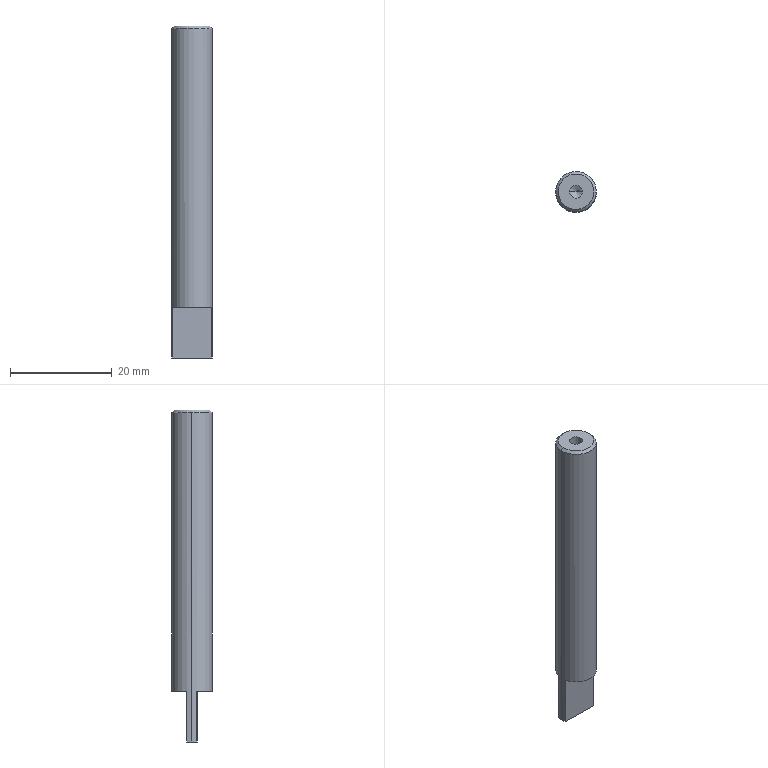Component | SolidWorks | 002MaterialPickingModuleA-1_004SidePlugModule-1_J-010-1 | 1 solid | 14 faces | box 8 x 8 x 65.25 mm | volume 2894 mm3 | plane 6 | cone 4 | cylinder 4 | commonest cylinder face diameters 2.5 x2 8 x2 | material 45
build123d program:
from build123d import *

# Parameters (mm, degrees)
SKETCH1_R             = 4
BOSS_EXTRUDE1_DEPTH   = 65.25
CUT_EXTRUDE1_START    = -10
CUT_EXTRUDE1_DEPTH    = 10
M3_TAPPED_HOLE1_D     = 2.5
M3_TAPPED_HOLE1_DEPTH = 7.5
M3_TAPPED_HOLE1_TIP   = 0.7511
CHAMFER1_SIZE         = 0.5


with BuildPart() as part:
    # Sketch1 → Boss-Extrude1 (new body)
    with BuildSketch(Plane.XY):
        Circle(SKETCH1_R)
    extrude(amount=BOSS_EXTRUDE1_DEPTH)

    # Sketch2 → Cut-Extrude1 (cut)
    with BuildSketch(Plane.XY.offset(65.25).offset(CUT_EXTRUDE1_START)):
        with BuildLine():
            Line((3.873, -1), (-3.873, -1))
            ThreePointArc((-3.873, -1), (0, -4), (3.873, -1))
        make_face()
        with BuildLine():
            Line((3.873, 1), (-3.873, 1))
            ThreePointArc((-3.873, 1), (0, 4), (3.873, 1))
        make_face()
    extrude(amount=CUT_EXTRUDE1_DEPTH, mode=Mode.SUBTRACT)

    # M3 Tapped Hole1
    with Locations(Plane(origin=(0, 0, 0), x_dir=(-1, 0, 0), z_dir=(0, 0, -1))):
        with Locations((0, 0)):
            Hole(M3_TAPPED_HOLE1_D / 2, depth=M3_TAPPED_HOLE1_DEPTH)
            with Locations((0, 0, -(M3_TAPPED_HOLE1_DEPTH + M3_TAPPED_HOLE1_TIP / 2))):  # 118° drill point
                Cone(0, M3_TAPPED_HOLE1_D / 2, M3_TAPPED_HOLE1_TIP, mode=Mode.SUBTRACT)

    # Chamfer1
    chamfer1_edges = [part.edges().sort_by_distance(p)[0] for p in [
        (-4, 0, 0),
    ]]
    chamfer(chamfer1_edges, length=CHAMFER1_SIZE)


solid = part.part

# Placed as in the assembly
solid = solid.moved(Location((70.325, 296.019, 469.581), (-180, 0, -179.039)))
STEP:
#1=CARTESIAN_POINT('',(2.906,11.652,18.487));
#2=VERTEX_POINT('',#1);
#3=CARTESIAN_POINT('',(2.631,11.657,18.487));
#4=VERTEX_POINT('',#3);
#5=CARTESIAN_POINT('',(2.769,11.654,18.487));
#6=DIRECTION('',(0.,0.,1.));
#7=DIRECTION('',(-0.9999,0.01678,0.));
#8=AXIS2_PLACEMENT_3D('',#5,#6,#7);
#9=CIRCLE('',#8,0.1378);
#10=EDGE_CURVE('',#2,#4,#9,.T.);
#11=ORIENTED_EDGE('',*,*,#10,.F.);
#12=CARTESIAN_POINT('',(2.926,11.652,18.468));
#13=VERTEX_POINT('',#12);
#14=CARTESIAN_POINT('',(2.926,11.652,18.468));
#15=DIRECTION('',(0.707,-0.01187,-0.7071));
#16=VECTOR('',#15,39.37);
#17=LINE('',#14,#16);
#18=EDGE_CURVE('',#2,#13,#17,.T.);
#19=ORIENTED_EDGE('',*,*,#18,.T.);
#20=CARTESIAN_POINT('',(2.611,11.657,18.468));
#21=VERTEX_POINT('',#20);
#22=CARTESIAN_POINT('',(2.769,11.654,18.468));
#23=DIRECTION('',(0.,0.,-1.));
#24=DIRECTION('',(-0.9999,0.01678,0.));
#25=AXIS2_PLACEMENT_3D('',#22,#23,#24);
#26=CIRCLE('',#25,0.1575);
#27=EDGE_CURVE('',#21,#13,#26,.T.);
#28=ORIENTED_EDGE('',*,*,#27,.F.);
#29=CARTESIAN_POINT('',(2.611,11.657,18.468));
#30=DIRECTION('',(-0.707,0.01187,-0.7071));
#31=VECTOR('',#30,39.37);
#32=LINE('',#29,#31);
#33=EDGE_CURVE('',#4,#21,#32,.T.);
#34=ORIENTED_EDGE('',*,*,#33,.F.);
#35=EDGE_LOOP('',(#11,#19,#28,#34));
#36=FACE_OUTER_BOUND('',#35,.T.);
#37=CARTESIAN_POINT('',(2.769,11.654,18.468));
#38=DIRECTION('',(0.,0.,-1.));
#39=DIRECTION('',(-0.9999,0.01678,0.));
#40=AXIS2_PLACEMENT_3D('',#37,#38,#39);
#41=CONICAL_SURFACE('',#40,0.1575,0.7854);
#42=ADVANCED_FACE('',(#36),#41,.T.);
#43=CARTESIAN_POINT('',(2.719,11.655,18.192));
#44=VERTEX_POINT('',#43);
#45=CARTESIAN_POINT('',(2.818,11.653,18.192));
#46=VERTEX_POINT('',#45);
#47=CARTESIAN_POINT('',(2.769,11.654,18.192));
#48=DIRECTION('',(0.,0.,1.));
#49=DIRECTION('',(0.9999,-0.01678,0.));
#50=AXIS2_PLACEMENT_3D('',#47,#48,#49);
#51=CIRCLE('',#50,0.04921);
#52=EDGE_CURVE('',#44,#46,#51,.T.);
#53=ORIENTED_EDGE('',*,*,#52,.F.);
#54=CARTESIAN_POINT('',(2.719,11.655,18.487));
#55=VERTEX_POINT('',#54);
#56=CARTESIAN_POINT('',(2.719,11.655,18.487));
#57=DIRECTION('',(0.,0.,1.));
#58=VECTOR('',#57,39.37);
#59=LINE('',#56,#58);
#60=EDGE_CURVE('',#44,#55,#59,.T.);
#61=ORIENTED_EDGE('',*,*,#60,.T.);
#62=CARTESIAN_POINT('',(2.818,11.653,18.487));
#63=VERTEX_POINT('',#62);
#64=CARTESIAN_POINT('',(2.769,11.654,18.487));
#65=DIRECTION('',(0.,0.,1.));
#66=DIRECTION('',(0.9999,-0.01678,0.));
#67=AXIS2_PLACEMENT_3D('',#64,#65,#66);
#68=CIRCLE('',#67,0.04921);
#69=EDGE_CURVE('',#55,#63,#68,.T.);
#70=ORIENTED_EDGE('',*,*,#69,.T.);
#71=CARTESIAN_POINT('',(2.818,11.653,18.487));
#72=DIRECTION('',(0.,0.,1.));
#73=VECTOR('',#72,39.37);
#74=LINE('',#71,#73);
#75=EDGE_CURVE('',#46,#63,#74,.T.);
#76=ORIENTED_EDGE('',*,*,#75,.F.);
#77=EDGE_LOOP('',(#53,#61,#70,#76));
#78=FACE_OUTER_BOUND('',#77,.T.);
#79=CARTESIAN_POINT('',(2.769,11.654,18.487));
#80=DIRECTION('',(0.,0.,1.));
#81=DIRECTION('',(0.9999,-0.01678,0.));
#82=AXIS2_PLACEMENT_3D('',#79,#80,#81);
#83=CYLINDRICAL_SURFACE('',#82,0.04921);
#84=ADVANCED_FACE('',(#78),#83,.F.);
#85=CARTESIAN_POINT('',(2.769,11.654,18.163));
#86=VERTEX_POINT('',#85);
#87=CARTESIAN_POINT('',(2.818,11.653,18.192));
#88=DIRECTION('',(0.857,-0.01438,0.515));
#89=VECTOR('',#88,39.37);
#90=LINE('',#87,#89);
#91=EDGE_CURVE('',#86,#46,#90,.T.);
#92=ORIENTED_EDGE('',*,*,#91,.F.);
#93=CARTESIAN_POINT('',(2.719,11.655,18.192));
#94=DIRECTION('',(-0.857,0.01438,0.515));
#95=VECTOR('',#94,39.37);
#96=LINE('',#93,#95);
#97=EDGE_CURVE('',#86,#44,#96,.T.);
#98=ORIENTED_EDGE('',*,*,#97,.T.);
#99=ORIENTED_EDGE('',*,*,#52,.T.);
#100=EDGE_LOOP('',(#92,#98,#99));
#101=FACE_OUTER_BOUND('',#100,.T.);
#102=CARTESIAN_POINT('',(2.769,11.654,18.192));
#103=DIRECTION('',(0.,0.,1.));
#104=DIRECTION('',(0.9999,-0.01678,0.));
#105=AXIS2_PLACEMENT_3D('',#102,#103,#104);
#106=CONICAL_SURFACE('',#105,0.04921,1.03);
#107=ADVANCED_FACE('',(#101),#106,.F.);
#108=CARTESIAN_POINT('',(2.611,11.657,15.919));
#109=VERTEX_POINT('',#108);
#110=CARTESIAN_POINT('',(2.617,11.696,15.919));
#111=VERTEX_POINT('',#110);
#112=CARTESIAN_POINT('',(2.769,11.654,15.919));
#113=DIRECTION('',(0.,0.,-1.));
#114=DIRECTION('',(-0.9999,0.01678,0.));
#115=AXIS2_PLACEMENT_3D('',#112,#113,#114);
#116=CIRCLE('',#115,0.1575);
#117=EDGE_CURVE('',#109,#111,#116,.T.);
#118=ORIENTED_EDGE('',*,*,#117,.F.);
#119=CARTESIAN_POINT('',(2.611,11.657,15.919));
#120=DIRECTION('',(0.,0.,1.));
#121=VECTOR('',#120,39.37);
#122=LINE('',#119,#121);
#123=EDGE_CURVE('',#109,#21,#122,.T.);
#124=ORIENTED_EDGE('',*,*,#123,.T.);
#125=ORIENTED_EDGE('',*,*,#27,.T.);
#126=CARTESIAN_POINT('',(2.926,11.652,15.919));
#127=VERTEX_POINT('',#126);
#128=CARTESIAN_POINT('',(2.926,11.652,15.919));
#129=DIRECTION('',(0.,0.,1.));
#130=VECTOR('',#129,39.37);
#131=LINE('',#128,#130);
#132=EDGE_CURVE('',#127,#13,#131,.T.);
#133=ORIENTED_EDGE('',*,*,#132,.F.);
#134=CARTESIAN_POINT('',(2.922,11.691,15.919));
#135=VERTEX_POINT('',#134);
#136=CARTESIAN_POINT('',(2.769,11.654,15.919));
#137=DIRECTION('',(0.,0.,-1.));
#138=DIRECTION('',(-0.9999,0.01678,0.));
#139=AXIS2_PLACEMENT_3D('',#136,#137,#138);
#140=CIRCLE('',#139,0.1575);
#141=EDGE_CURVE('',#135,#127,#140,.T.);
#142=ORIENTED_EDGE('',*,*,#141,.F.);
#143=CARTESIAN_POINT('',(2.922,11.691,16.312));
#144=VERTEX_POINT('',#143);
#145=CARTESIAN_POINT('',(2.922,11.691,16.312));
#146=DIRECTION('',(0.,0.,-1.));
#147=VECTOR('',#146,39.37);
#148=LINE('',#145,#147);
#149=EDGE_CURVE('',#144,#135,#148,.T.);
#150=ORIENTED_EDGE('',*,*,#149,.F.);
#151=CARTESIAN_POINT('',(2.617,11.696,16.312));
#152=VERTEX_POINT('',#151);
#153=CARTESIAN_POINT('',(2.769,11.654,16.312));
#154=DIRECTION('',(0.,0.,-1.));
#155=DIRECTION('',(-0.9999,0.01678,0.));
#156=AXIS2_PLACEMENT_3D('',#153,#154,#155);
#157=CIRCLE('',#156,0.1575);
#158=EDGE_CURVE('',#152,#144,#157,.T.);
#159=ORIENTED_EDGE('',*,*,#158,.F.);
#160=CARTESIAN_POINT('',(2.617,11.696,16.312));
#161=DIRECTION('',(0.,0.,-1.));
#162=VECTOR('',#161,39.37);
#163=LINE('',#160,#162);
#164=EDGE_CURVE('',#152,#111,#163,.T.);
#165=ORIENTED_EDGE('',*,*,#164,.T.);
#166=EDGE_LOOP('',(#118,#124,#125,#133,#142,#150,#159,#165));
#167=FACE_OUTER_BOUND('',#166,.T.);
#168=CARTESIAN_POINT('',(2.769,11.654,15.919));
#169=DIRECTION('',(0.,0.,1.));
#170=DIRECTION('',(0.9999,-0.01678,0.));
#171=AXIS2_PLACEMENT_3D('',#168,#169,#170);
#172=CYLINDRICAL_SURFACE('',#171,0.1575);
#173=ADVANCED_FACE('',(#167),#172,.T.);
#174=ORIENTED_EDGE('',*,*,#123,.F.);
#175=CARTESIAN_POINT('',(2.616,11.617,15.919));
#176=VERTEX_POINT('',#175);
#177=CARTESIAN_POINT('',(2.769,11.654,15.919));
#178=DIRECTION('',(0.,0.,-1.));
#179=DIRECTION('',(-0.9999,0.01678,0.));
#180=AXIS2_PLACEMENT_3D('',#177,#178,#179);
#181=CIRCLE('',#180,0.1575);
#182=EDGE_CURVE('',#176,#109,#181,.T.);
#183=ORIENTED_EDGE('',*,*,#182,.F.);
#184=CARTESIAN_POINT('',(2.616,11.617,16.312));
#185=VERTEX_POINT('',#184);
#186=CARTESIAN_POINT('',(2.616,11.617,16.312));
#187=DIRECTION('',(0.,0.,-1.));
#188=VECTOR('',#187,39.37);
#189=LINE('',#186,#188);
#190=EDGE_CURVE('',#185,#176,#189,.T.);
#191=ORIENTED_EDGE('',*,*,#190,.F.);
#192=CARTESIAN_POINT('',(2.92,11.612,16.312));
#193=VERTEX_POINT('',#192);
#194=CARTESIAN_POINT('',(2.769,11.654,16.312));
#195=DIRECTION('',(0.,0.,-1.));
#196=DIRECTION('',(-0.9999,0.01678,0.));
#197=AXIS2_PLACEMENT_3D('',#194,#195,#196);
#198=CIRCLE('',#197,0.1575);
#199=EDGE_CURVE('',#193,#185,#198,.T.);
#200=ORIENTED_EDGE('',*,*,#199,.F.);
#201=CARTESIAN_POINT('',(2.92,11.612,15.919));
#202=VERTEX_POINT('',#201);
#203=CARTESIAN_POINT('',(2.92,11.612,16.312));
#204=DIRECTION('',(0.,0.,-1.));
#205=VECTOR('',#204,39.37);
#206=LINE('',#203,#205);
#207=EDGE_CURVE('',#193,#202,#206,.T.);
#208=ORIENTED_EDGE('',*,*,#207,.T.);
#209=CARTESIAN_POINT('',(2.769,11.654,15.919));
#210=DIRECTION('',(0.,0.,-1.));
#211=DIRECTION('',(-0.9999,0.01678,0.));
#212=AXIS2_PLACEMENT_3D('',#209,#210,#211);
#213=CIRCLE('',#212,0.1575);
#214=EDGE_CURVE('',#127,#202,#213,.T.);
#215=ORIENTED_EDGE('',*,*,#214,.F.);
#216=ORIENTED_EDGE('',*,*,#132,.T.);
#217=CARTESIAN_POINT('',(2.769,11.654,18.468));
#218=DIRECTION('',(0.,0.,-1.));
#219=DIRECTION('',(-0.9999,0.01678,0.));
#220=AXIS2_PLACEMENT_3D('',#217,#218,#219);
#221=CIRCLE('',#220,0.1575);
#222=EDGE_CURVE('',#13,#21,#221,.T.);
#223=ORIENTED_EDGE('',*,*,#222,.T.);
#224=EDGE_LOOP('',(#174,#183,#191,#200,#208,#215,#216,#223));
#225=FACE_OUTER_BOUND('',#224,.T.);
#226=CARTESIAN_POINT('',(2.769,11.654,15.919));
#227=DIRECTION('',(0.,0.,1.));
#228=DIRECTION('',(0.9999,-0.01678,0.));
#229=AXIS2_PLACEMENT_3D('',#226,#227,#228);
#230=CYLINDRICAL_SURFACE('',#229,0.1575);
#231=ADVANCED_FACE('',(#225),#230,.T.);
#232=CARTESIAN_POINT('',(2.616,11.617,15.919));
#233=DIRECTION('',(0.9999,-0.01678,0.));
#234=VECTOR('',#233,39.37);
#235=LINE('',#232,#234);
#236=EDGE_CURVE('',#176,#202,#235,.T.);
#237=ORIENTED_EDGE('',*,*,#236,.F.);
#238=ORIENTED_EDGE('',*,*,#182,.T.);
#239=ORIENTED_EDGE('',*,*,#117,.T.);
#240=CARTESIAN_POINT('',(2.617,11.696,15.919));
#241=DIRECTION('',(-0.9999,0.01678,0.));
#242=VECTOR('',#241,39.37);
#243=LINE('',#240,#242);
#244=EDGE_CURVE('',#135,#111,#243,.T.);
#245=ORIENTED_EDGE('',*,*,#244,.F.);
#246=ORIENTED_EDGE('',*,*,#141,.T.);
#247=ORIENTED_EDGE('',*,*,#214,.T.);
#248=EDGE_LOOP('',(#237,#238,#239,#245,#246,#247));
#249=FACE_OUTER_BOUND('',#248,.T.);
#250=CARTESIAN_POINT('',(2.769,11.654,15.919));
#251=DIRECTION('',(0.,0.,-1.));
#252=DIRECTION('',(-0.9999,0.01678,0.));
#253=AXIS2_PLACEMENT_3D('',#250,#251,#252);
#254=PLANE('',#253);
#255=ADVANCED_FACE('',(#249),#254,.T.);
#256=CARTESIAN_POINT('',(2.769,11.654,18.487));
#257=DIRECTION('',(0.,0.,1.));
#258=DIRECTION('',(-0.9999,0.01678,0.));
#259=AXIS2_PLACEMENT_3D('',#256,#257,#258);
#260=CIRCLE('',#259,0.1378);
#261=EDGE_CURVE('',#4,#2,#260,.T.);
#262=ORIENTED_EDGE('',*,*,#261,.T.);
#263=ORIENTED_EDGE('',*,*,#10,.T.);
#264=EDGE_LOOP('',(#262,#263));
#265=FACE_OUTER_BOUND('',#264,.T.);
#266=CARTESIAN_POINT('',(2.769,11.654,18.487));
#267=DIRECTION('',(0.,0.,1.));
#268=DIRECTION('',(0.9999,-0.01678,0.));
#269=AXIS2_PLACEMENT_3D('',#266,#267,#268);
#270=CIRCLE('',#269,0.04921);
#271=EDGE_CURVE('',#63,#55,#270,.T.);
#272=ORIENTED_EDGE('',*,*,#271,.F.);
#273=ORIENTED_EDGE('',*,*,#69,.F.);
#274=EDGE_LOOP('',(#272,#273));
#275=FACE_BOUND('',#274,.T.);
#276=CARTESIAN_POINT('',(2.769,11.654,18.487));
#277=DIRECTION('',(0.,0.,-1.));
#278=DIRECTION('',(-0.9999,0.01678,0.));
#279=AXIS2_PLACEMENT_3D('',#276,#277,#278);
#280=PLANE('',#279);
#281=ADVANCED_FACE('',(#265,#275),#280,.F.);
#282=ORIENTED_EDGE('',*,*,#244,.T.);
#283=ORIENTED_EDGE('',*,*,#164,.F.);
#284=CARTESIAN_POINT('',(2.617,11.696,16.312));
#285=DIRECTION('',(-0.9999,0.01678,0.));
#286=VECTOR('',#285,39.37);
#287=LINE('',#284,#286);
#288=EDGE_CURVE('',#144,#152,#287,.T.);
#289=ORIENTED_EDGE('',*,*,#288,.F.);
#290=ORIENTED_EDGE('',*,*,#149,.T.);
#291=EDGE_LOOP('',(#282,#283,#289,#290));
#292=FACE_OUTER_BOUND('',#291,.T.);
#293=CARTESIAN_POINT('',(2.617,11.696,16.312));
#294=DIRECTION('',(-0.01678,-0.9999,0.));
#295=DIRECTION('',(0.,0.,1.));
#296=AXIS2_PLACEMENT_3D('',#293,#294,#295);
#297=PLANE('',#296);
#298=ADVANCED_FACE('',(#292),#297,.F.);
#299=ORIENTED_EDGE('',*,*,#158,.T.);
#300=ORIENTED_EDGE('',*,*,#288,.T.);
#301=EDGE_LOOP('',(#299,#300));
#302=FACE_OUTER_BOUND('',#301,.T.);
#303=CARTESIAN_POINT('',(2.769,11.654,16.312));
#304=DIRECTION('',(0.,0.,-1.));
#305=DIRECTION('',(-0.9999,0.01678,0.));
#306=AXIS2_PLACEMENT_3D('',#303,#304,#305);
#307=PLANE('',#306);
#308=ADVANCED_FACE('',(#302),#307,.T.);
#309=ORIENTED_EDGE('',*,*,#236,.T.);
#310=ORIENTED_EDGE('',*,*,#207,.F.);
#311=CARTESIAN_POINT('',(2.616,11.617,16.312));
#312=DIRECTION('',(0.9999,-0.01678,0.));
#313=VECTOR('',#312,39.37);
#314=LINE('',#311,#313);
#315=EDGE_CURVE('',#185,#193,#314,.T.);
#316=ORIENTED_EDGE('',*,*,#315,.F.);
#317=ORIENTED_EDGE('',*,*,#190,.T.);
#318=EDGE_LOOP('',(#309,#310,#316,#317));
#319=FACE_OUTER_BOUND('',#318,.T.);
#320=CARTESIAN_POINT('',(2.616,11.617,16.312));
#321=DIRECTION('',(0.01678,0.9999,0.));
#322=DIRECTION('',(0.,0.,-1.));
#323=AXIS2_PLACEMENT_3D('',#320,#321,#322);
#324=PLANE('',#323);
#325=ADVANCED_FACE('',(#319),#324,.F.);
#326=ORIENTED_EDGE('',*,*,#199,.T.);
#327=ORIENTED_EDGE('',*,*,#315,.T.);
#328=EDGE_LOOP('',(#326,#327));
#329=FACE_OUTER_BOUND('',#328,.T.);
#330=CARTESIAN_POINT('',(2.769,11.654,16.312));
#331=DIRECTION('',(0.,0.,-1.));
#332=DIRECTION('',(-0.9999,0.01678,0.));
#333=AXIS2_PLACEMENT_3D('',#330,#331,#332);
#334=PLANE('',#333);
#335=ADVANCED_FACE('',(#329),#334,.T.);
#336=ORIENTED_EDGE('',*,*,#97,.F.);
#337=ORIENTED_EDGE('',*,*,#91,.T.);
#338=CARTESIAN_POINT('',(2.769,11.654,18.192));
#339=DIRECTION('',(0.,0.,1.));
#340=DIRECTION('',(0.9999,-0.01678,0.));
#341=AXIS2_PLACEMENT_3D('',#338,#339,#340);
#342=CIRCLE('',#341,0.04921);
#343=EDGE_CURVE('',#46,#44,#342,.T.);
#344=ORIENTED_EDGE('',*,*,#343,.T.);
#345=EDGE_LOOP('',(#336,#337,#344));
#346=FACE_OUTER_BOUND('',#345,.T.);
#347=CARTESIAN_POINT('',(2.769,11.654,18.192));
#348=DIRECTION('',(0.,0.,1.));
#349=DIRECTION('',(0.9999,-0.01678,0.));
#350=AXIS2_PLACEMENT_3D('',#347,#348,#349);
#351=CONICAL_SURFACE('',#350,0.04921,1.03);
#352=ADVANCED_FACE('',(#346),#351,.F.);
#353=ORIENTED_EDGE('',*,*,#60,.F.);
#354=ORIENTED_EDGE('',*,*,#343,.F.);
#355=ORIENTED_EDGE('',*,*,#75,.T.);
#356=ORIENTED_EDGE('',*,*,#271,.T.);
#357=EDGE_LOOP('',(#353,#354,#355,#356));
#358=FACE_OUTER_BOUND('',#357,.T.);
#359=CARTESIAN_POINT('',(2.769,11.654,18.487));
#360=DIRECTION('',(0.,0.,1.));
#361=DIRECTION('',(0.9999,-0.01678,0.));
#362=AXIS2_PLACEMENT_3D('',#359,#360,#361);
#363=CYLINDRICAL_SURFACE('',#362,0.04921);
#364=ADVANCED_FACE('',(#358),#363,.F.);
#365=ORIENTED_EDGE('',*,*,#18,.F.);
#366=ORIENTED_EDGE('',*,*,#261,.F.);
#367=ORIENTED_EDGE('',*,*,#33,.T.);
#368=ORIENTED_EDGE('',*,*,#222,.F.);
#369=EDGE_LOOP('',(#365,#366,#367,#368));
#370=FACE_OUTER_BOUND('',#369,.T.);
#371=CARTESIAN_POINT('',(2.769,11.654,18.468));
#372=DIRECTION('',(0.,0.,-1.));
#373=DIRECTION('',(-0.9999,0.01678,0.));
#374=AXIS2_PLACEMENT_3D('',#371,#372,#373);
#375=CONICAL_SURFACE('',#374,0.1575,0.7854);
#376=ADVANCED_FACE('',(#370),#375,.T.);
#377=CLOSED_SHELL('',(#42,#84,#107,#173,#231,#255,#281,#298,#308,#325,#335,#352,#364,#376));
#378=MANIFOLD_SOLID_BREP('',#377);
#379=CARTESIAN_POINT('',(0.,0.,0.));
#380=DIRECTION('',(0.,0.,1.));
#381=DIRECTION('',(1.,0.,0.));
#382=AXIS2_PLACEMENT_3D('',#379,#380,#381);
#383=(LENGTH_UNIT()NAMED_UNIT(*)SI_UNIT($,.METRE.));
#384=LENGTH_MEASURE_WITH_UNIT(LENGTH_MEASURE(0.0254),#383);
#385=DIMENSIONAL_EXPONENTS(1.,0.,0.,0.,0.,0.,0.);
#386=(CONVERSION_BASED_UNIT('',#384)LENGTH_UNIT()NAMED_UNIT(#385));
#387=UNCERTAINTY_MEASURE_WITH_UNIT(LENGTH_MEASURE(0.00001),#386,'','');
#388=(NAMED_UNIT(*)PLANE_ANGLE_UNIT()SI_UNIT($,.RADIAN.));
#389=(NAMED_UNIT(*)SI_UNIT($,.STERADIAN.)SOLID_ANGLE_UNIT());
#390=(GEOMETRIC_REPRESENTATION_CONTEXT(3)GLOBAL_UNCERTAINTY_ASSIGNED_CONTEXT((#387))GLOBAL_UNIT_ASSIGNED_CONTEXT((#386,#388,#389))REPRESENTATION_CONTEXT('',''));
#391=ADVANCED_BREP_SHAPE_REPRESENTATION('',(#378,#382),#390);
#392=COLOUR_RGB('',0.7922,0.8196,0.9333);
#393=FILL_AREA_STYLE_COLOUR('',#392);
#394=FILL_AREA_STYLE('',(#393));
#395=SURFACE_STYLE_FILL_AREA(#394);
#396=SURFACE_SIDE_STYLE('',(#395));
#397=SURFACE_STYLE_USAGE(.BOTH.,#396);
#398=PRESENTATION_STYLE_ASSIGNMENT((#397));
#399=STYLED_ITEM('',(#398),#378);
#400=(LENGTH_UNIT()NAMED_UNIT(*)SI_UNIT($,.METRE.));
#401=LENGTH_MEASURE_WITH_UNIT(LENGTH_MEASURE(0.0254),#400);
#402=DIMENSIONAL_EXPONENTS(1.,0.,0.,0.,0.,0.,0.);
#403=(CONVERSION_BASED_UNIT('',#401)LENGTH_UNIT()NAMED_UNIT(#402));
#404=UNCERTAINTY_MEASURE_WITH_UNIT(LENGTH_MEASURE(0.00001),#403,'','');
#405=(NAMED_UNIT(*)PLANE_ANGLE_UNIT()SI_UNIT($,.RADIAN.));
#406=(NAMED_UNIT(*)SI_UNIT($,.STERADIAN.)SOLID_ANGLE_UNIT());
#407=(GEOMETRIC_REPRESENTATION_CONTEXT(3)GLOBAL_UNCERTAINTY_ASSIGNED_CONTEXT((#404))GLOBAL_UNIT_ASSIGNED_CONTEXT((#403,#405,#406))REPRESENTATION_CONTEXT('',''));
#408=MECHANICAL_DESIGN_GEOMETRIC_PRESENTATION_REPRESENTATION('',(#399),#407);
#409=PRESENTATION_LAYER_ASSIGNMENT('','',(#399));